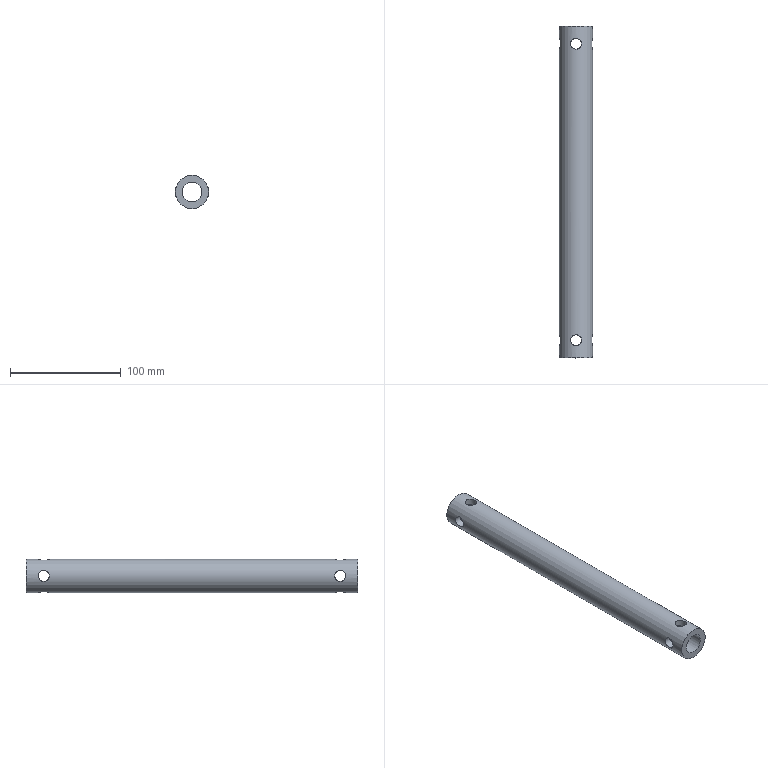Component | NX | CONNECTING_ROD_MODEL1 | 1 solid | 12 faces | volume 131853 mm3 | cylinder 10 | plane 2 | commonest cylinder face diameters 10 x8 30 x1 18 x1